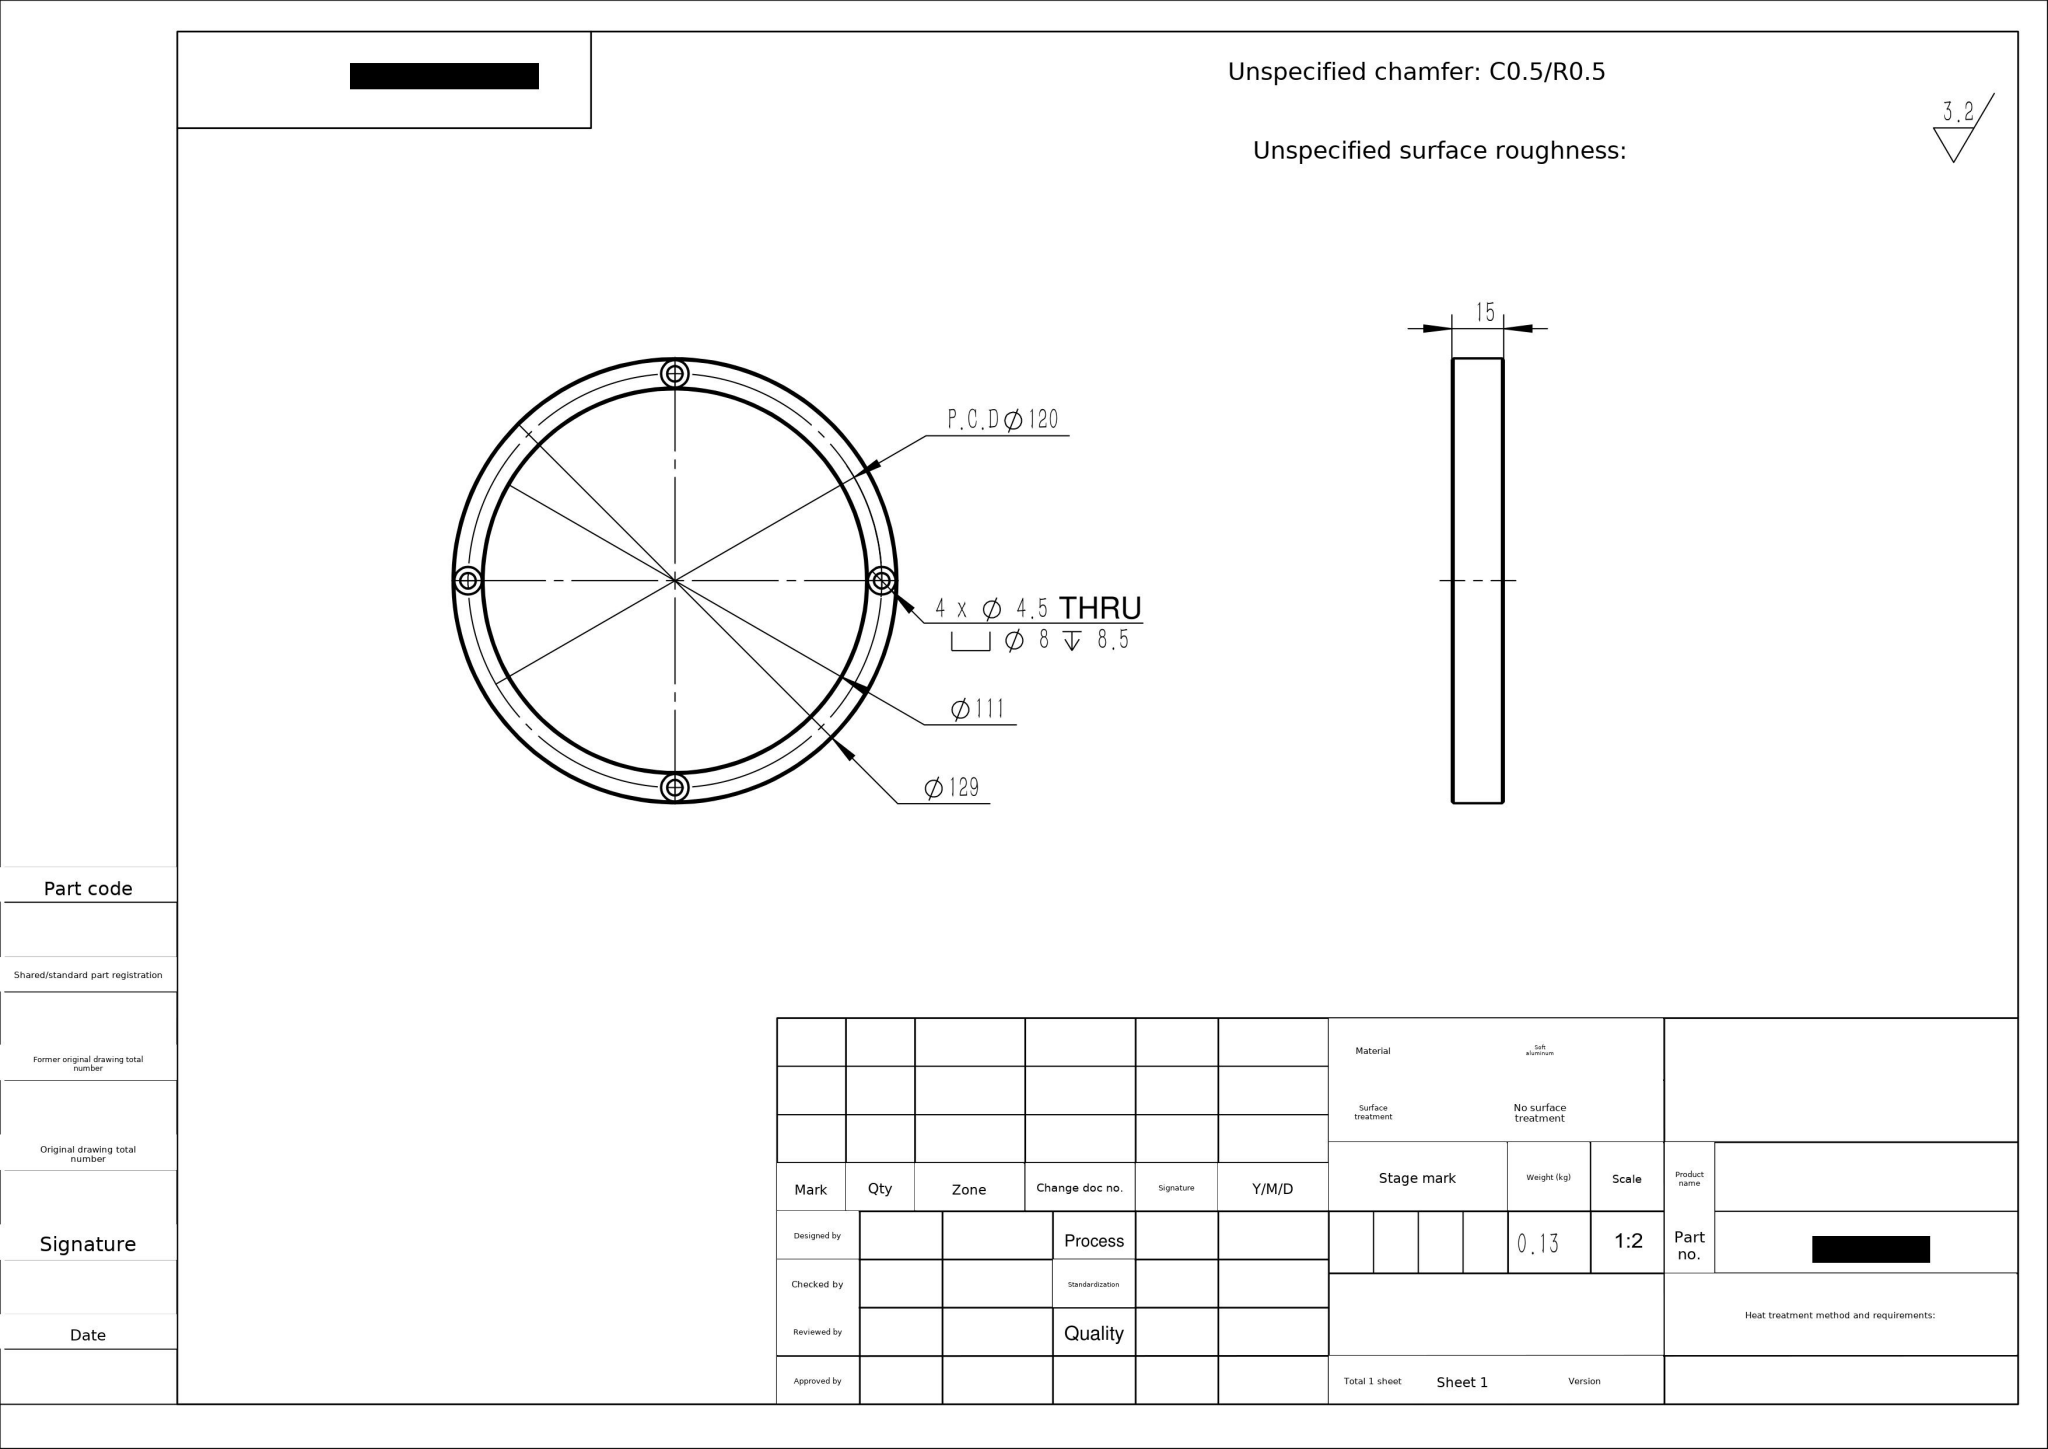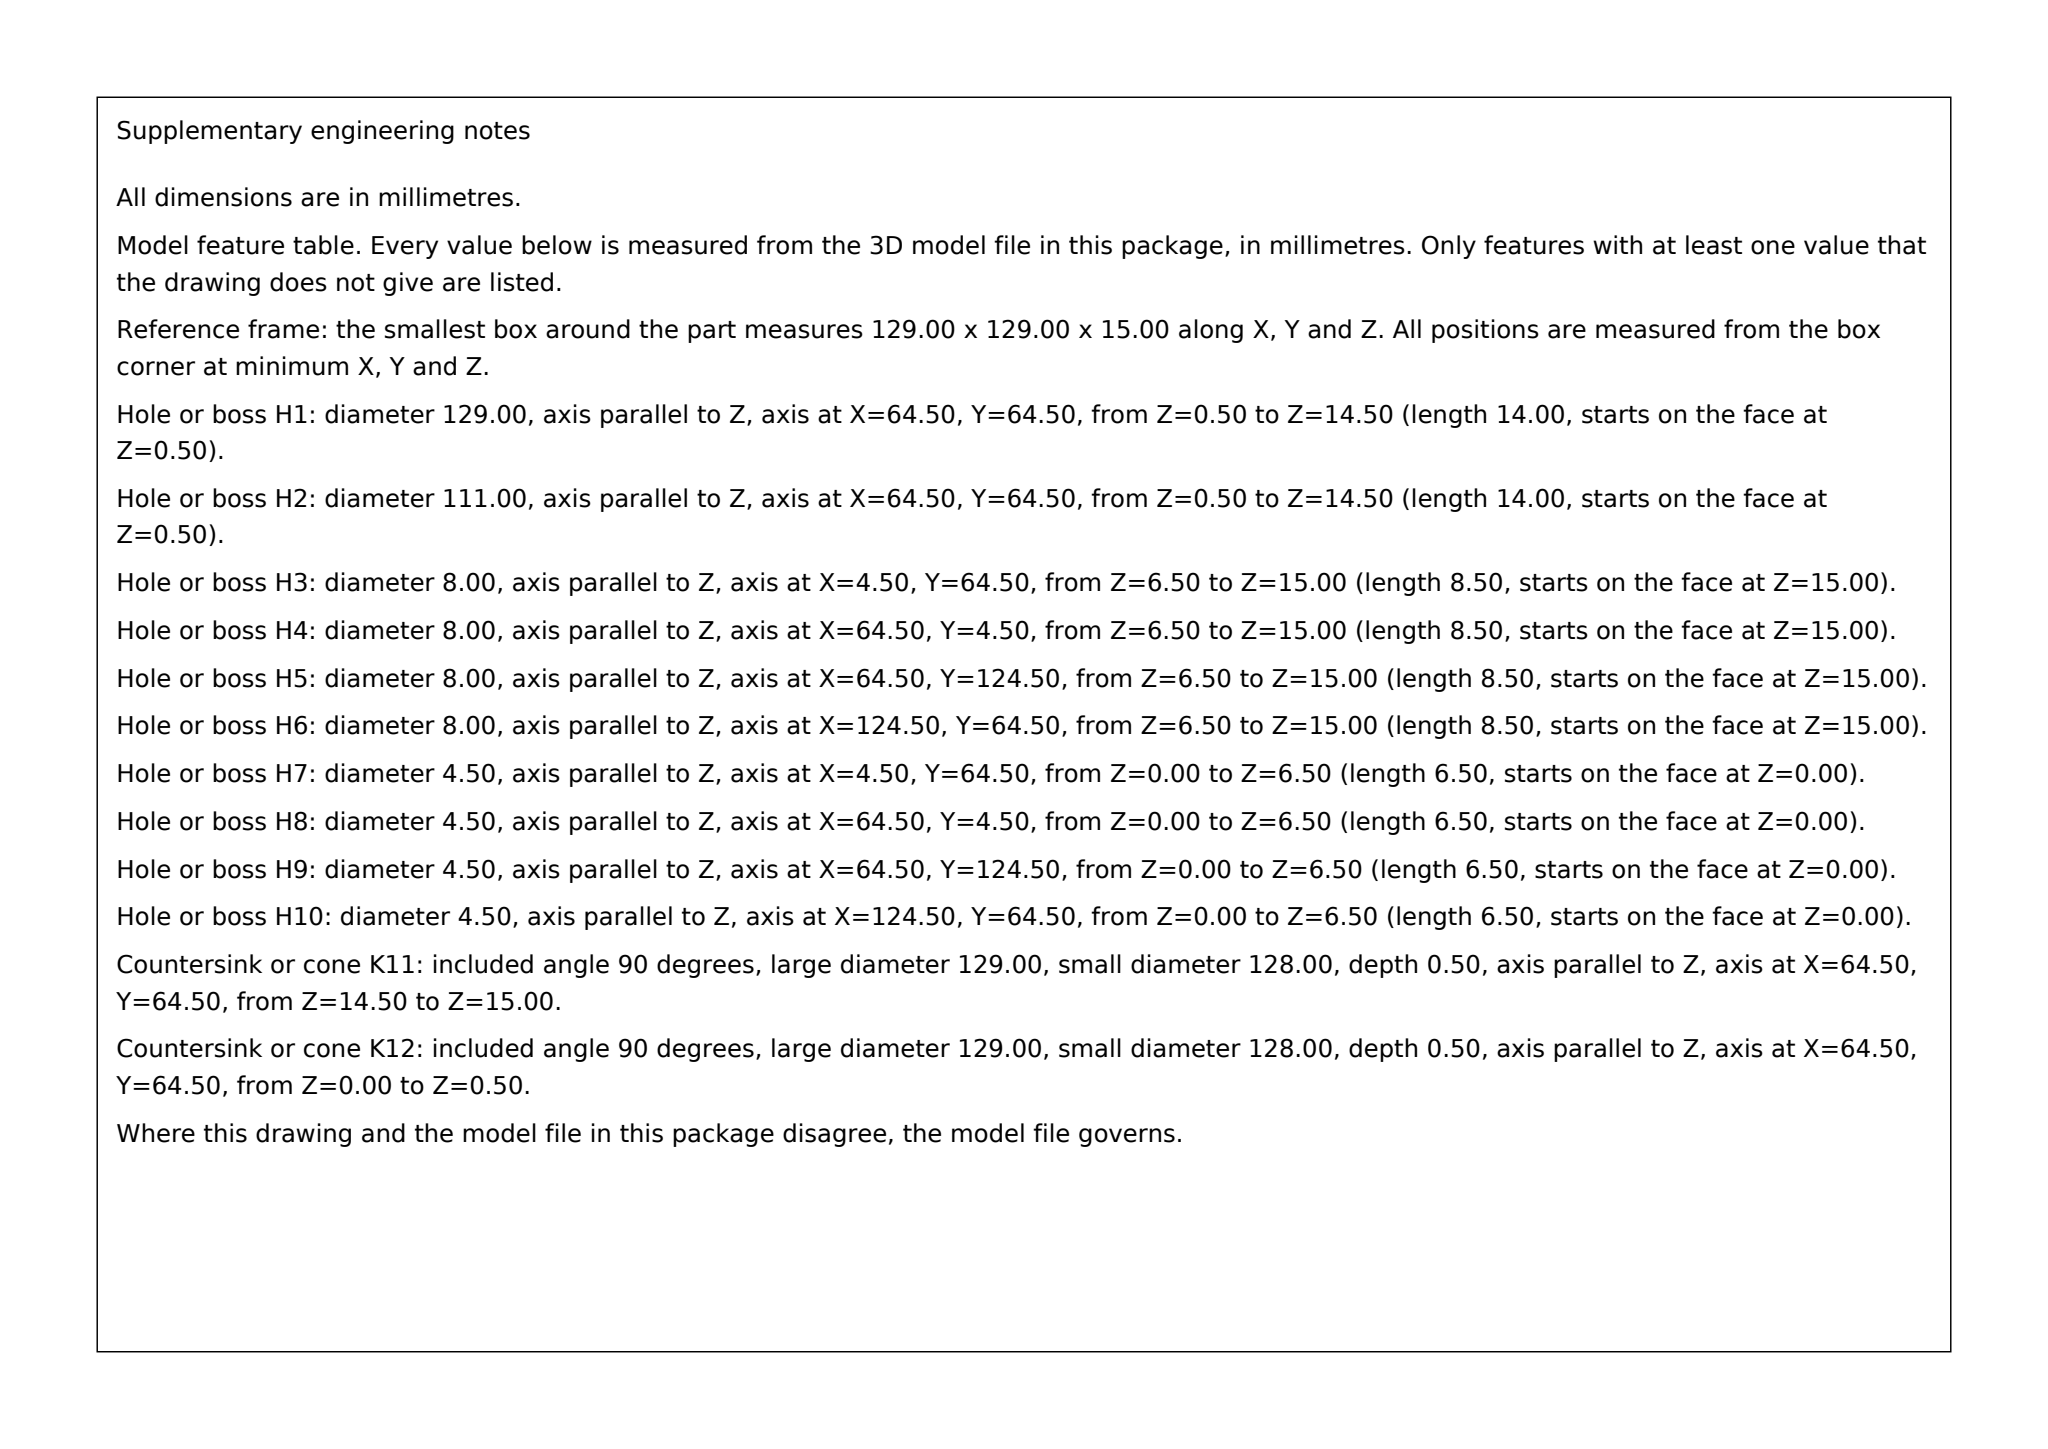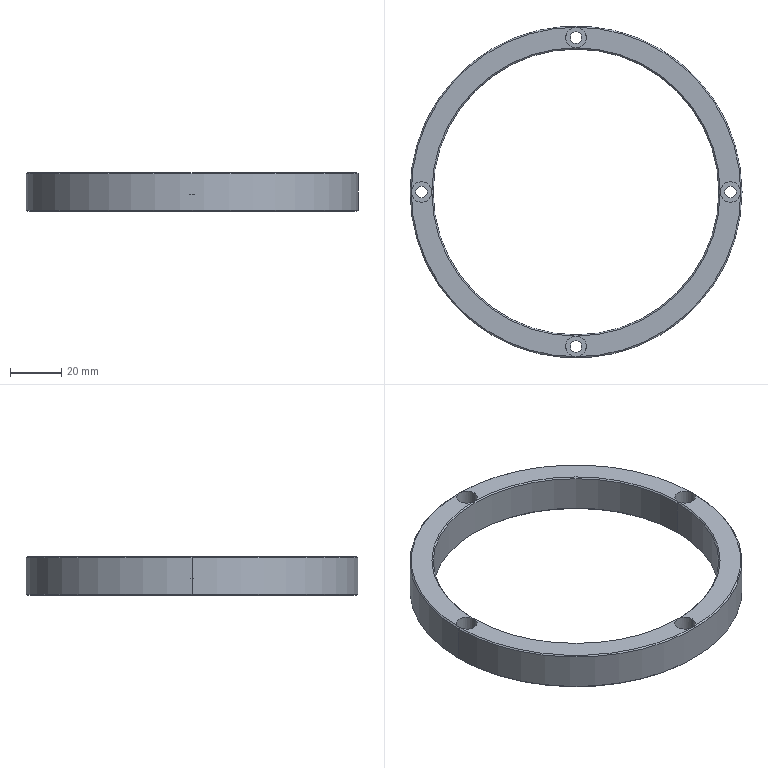Part | SolidWorks | mm | material Soft aluminum | 1 solid | 37 faces | box 129 x 129 x 15 mm | volume 48583 mm3 | cylinder 20 | plane 9 | cone 8 | commonest cylinder face diameters 8 x8 4.5 x8 111 x2 129 x2